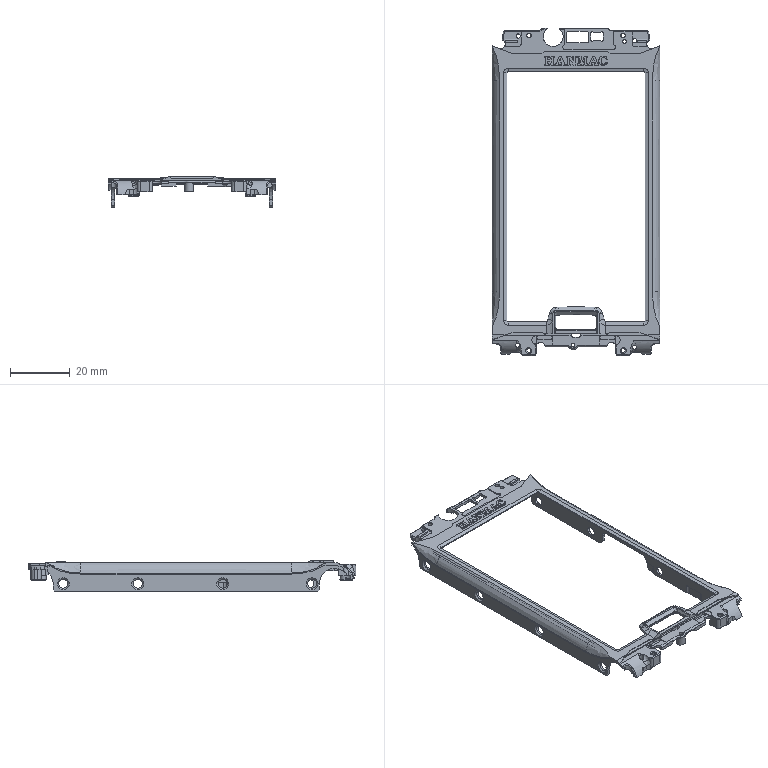CAM job | NX | mm | 3-axis | 1 set-up | 9 operations | part box 56 x 109.27 x 10.34
set-up 1
1. Planar Milling | Mill Mill5 D63 | PLANAR_MILL | path 216.273 mm | 0.1582 min
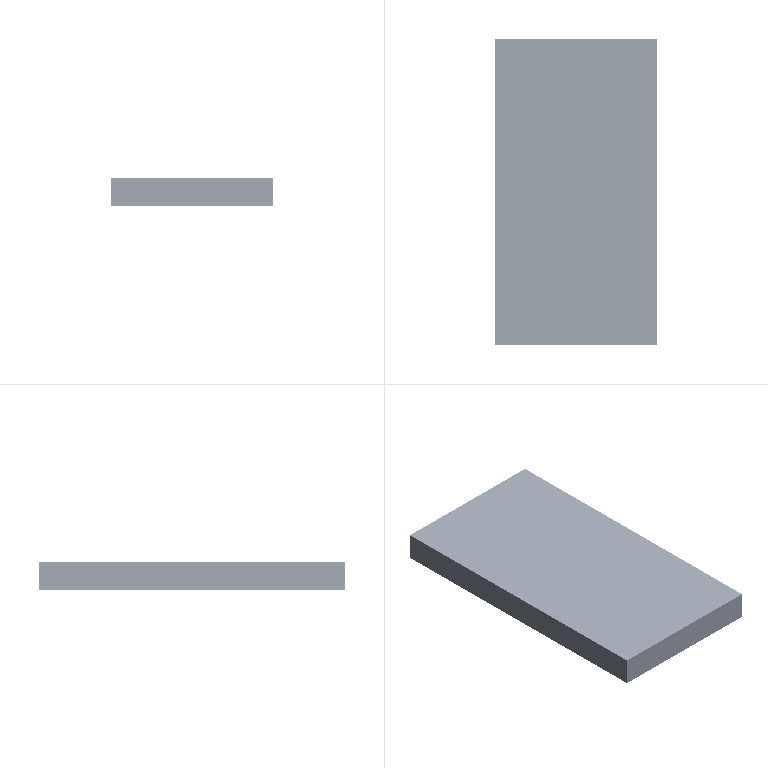2. Planar Milling | Mill Mill5 D12 | PLANAR_MILL_1 | path 1751.028 mm | 0.9817 min
3. Planar Milling | Mill Mill5 D12 | PLANAR_MILL_1_COPY | path 1550.81 mm | 0.9417 min
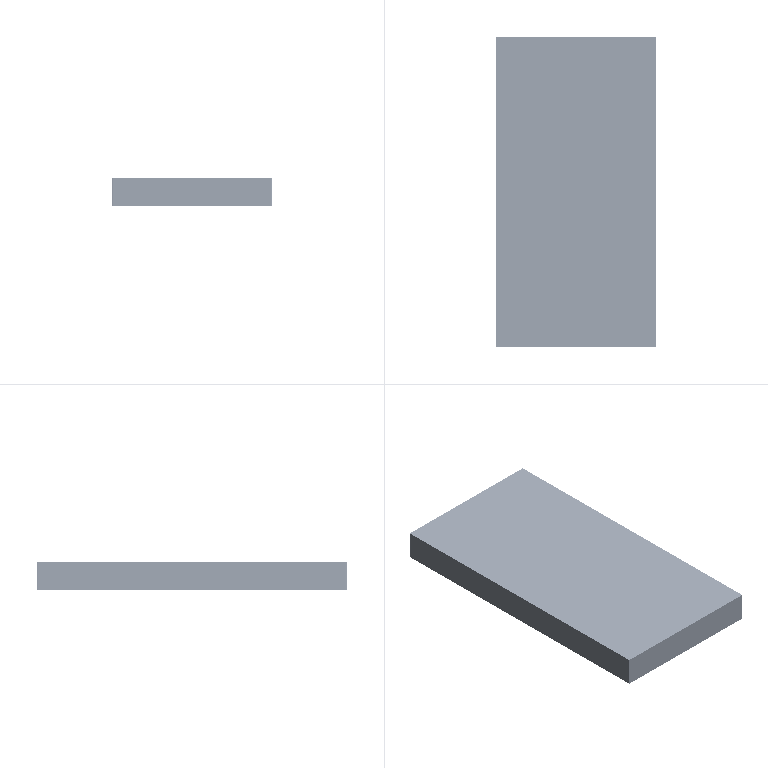4. Z-Level Milling | Mill Mill5 D12 | ZLEVEL_PROFILE | path 8917.385 mm | 18.625 min
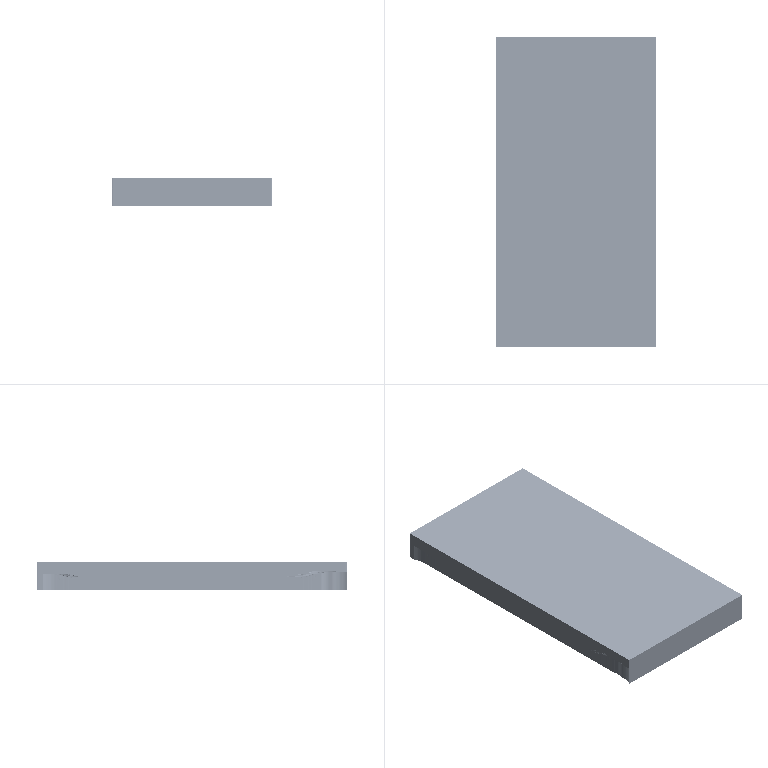5. Planar Milling | Mill Mill5 D12 | PLANAR_MILL_1_COPY_COPY | path 296.29 mm | 0.12 min
6. Cavity Milling | Mill Mill5 D12 | CAVITY_MILL | path 8075.76 mm | 17.615 min
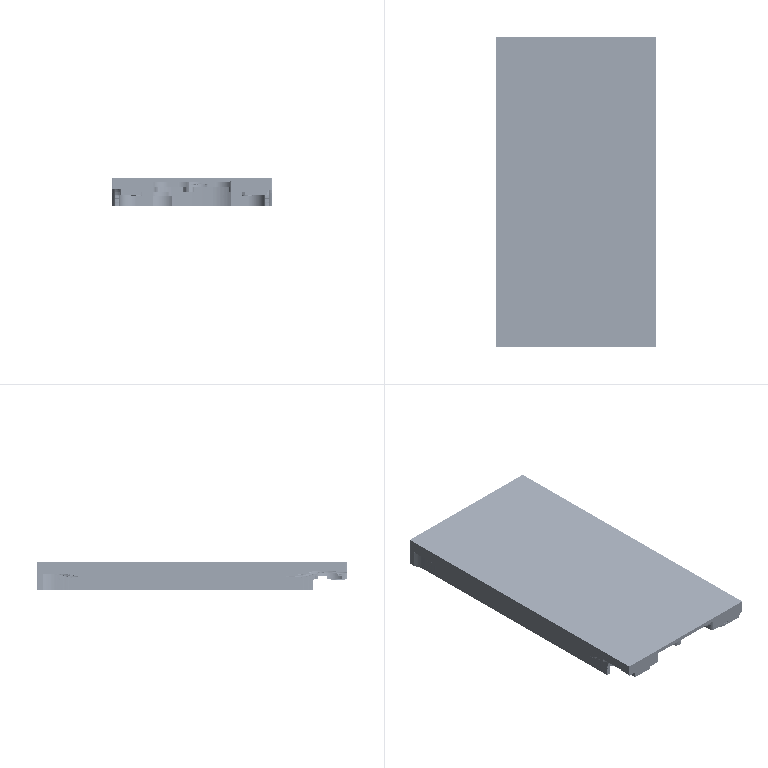7. Cavity Milling | Mill Mill5 D6 | CAVITY_MILL_COPY | path 7482.036 mm | 14.295 min
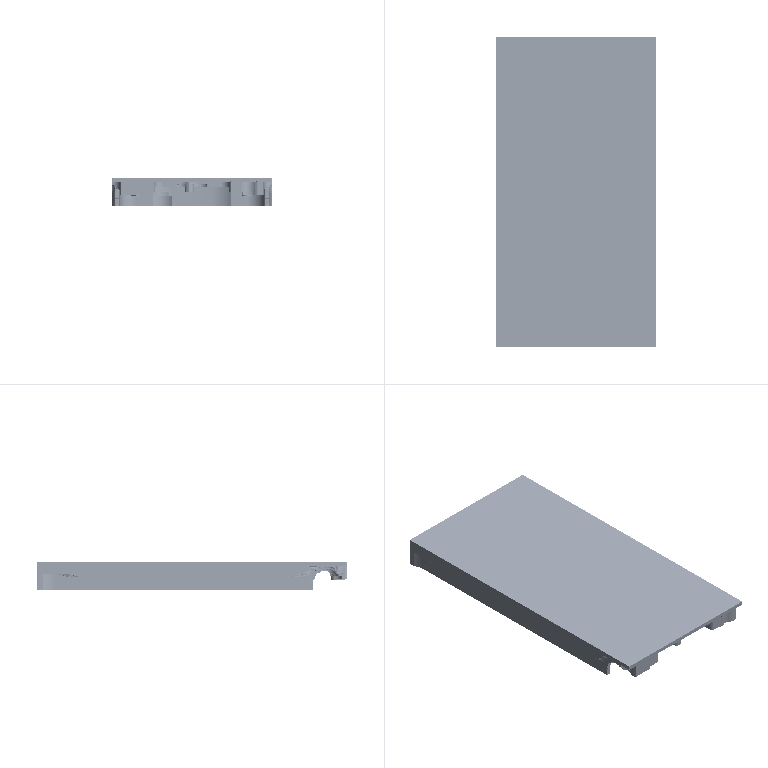8. Cavity Milling | Mill Mill5 D3 | CAVITY_MILL_COPY_COPY | path 6722.05 mm | 14.193 min
9. Planar Milling | Mill Mill5 D12 | SOLID_PROFILE_3D | path 190.577 mm | 0.6366 min